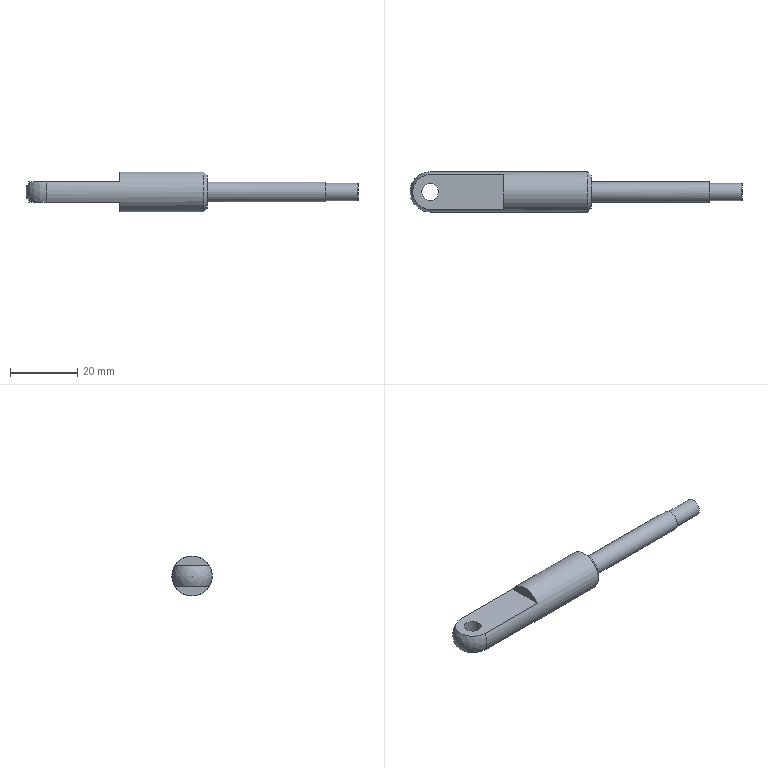Component | NX | SCREW_ROD | 1 solid | 14 faces | box 99 x 12 x 12 mm | volume 5834 mm3 | plane 7 | cylinder 4 | cone 2 | sphere 1 | commonest cylinder face diameters 12 x1 5 x1 6 x1 5.188 x1
STEP:
#1=CARTESIAN_POINT('',(0.,0.,0.));
#2=DIRECTION('',(0.,0.,1.));
#3=DIRECTION('',(1.,0.,0.));
#4=AXIS2_PLACEMENT_3D('',#1,#2,#3);
#5=CARTESIAN_POINT('',(22.3,-37.25,-16.5));
#6=VERTEX_POINT('',#5);
#7=CARTESIAN_POINT('',(22.3,-43.25,-16.5));
#8=DIRECTION('',(-1.,0.,0.));
#9=DIRECTION('',(0.,1.,0.));
#10=AXIS2_PLACEMENT_3D('',#7,#8,#9);
#11=CIRCLE('',#10,6.);
#12=CARTESIAN_POINT('',(-30.7,-43.25,-16.5));
#13=DIRECTION('',(1.,0.,0.));
#14=DIRECTION('',(0.,1.,0.));
#15=AXIS2_PLACEMENT_3D('',#12,#13,#14);
#16=CYLINDRICAL_SURFACE('',#15,6.);
#17=CARTESIAN_POINT('',(6.283,53.));
#18=DIRECTION('',(-1.,0.));
#19=VECTOR('',#18,1.);
#20=LINE('',#17,#19);
#21=(GEOMETRIC_REPRESENTATION_CONTEXT(2)PARAMETRIC_REPRESENTATION_CONTEXT()REPRESENTATION_CONTEXT('',''));
#22=DEFINITIONAL_REPRESENTATION('',(#20),#21);
#23=PCURVE('',#16,#22);
#24=CARTESIAN_POINT('',(23.3,-43.25,-16.5));
#25=DIRECTION('',(-1.,0.,0.));
#26=DIRECTION('',(0.,-1.,0.));
#27=AXIS2_PLACEMENT_3D('',#24,#25,#26);
#28=CONICAL_SURFACE('',#27,5.,0.7854);
#29=CARTESIAN_POINT('',(3.142,1.));
#30=DIRECTION('',(1.,0.));
#31=VECTOR('',#30,1.);
#32=LINE('',#29,#31);
#33=(GEOMETRIC_REPRESENTATION_CONTEXT(2)PARAMETRIC_REPRESENTATION_CONTEXT()REPRESENTATION_CONTEXT('',''));
#34=DEFINITIONAL_REPRESENTATION('',(#32),#33);
#35=PCURVE('',#28,#34);
#36=SURFACE_CURVE('',#11,(#23,#35),.PCURVE_S1.);
#37=EDGE_CURVE('',#6,#6,#36,.T.);
#38=ORIENTED_EDGE('',*,*,#37,.T.);
#39=CARTESIAN_POINT('',(-24.7,-37.25,-16.5));
#40=VERTEX_POINT('',#39);
#41=CARTESIAN_POINT('',(-24.7,-37.25,-16.5));
#42=CARTESIAN_POINT('',(22.3,-37.25,-16.5));
#43=B_SPLINE_CURVE_WITH_KNOTS('',1,(#41,#42),.UNSPECIFIED.,.F.,.F.,(2,2),(6.,53.),.PIECEWISE_BEZIER_KNOTS.);
#44=CARTESIAN_POINT('',(0.,0.));
#45=DIRECTION('',(0.,1.));
#46=VECTOR('',#45,1.);
#47=LINE('',#44,#46);
#48=(GEOMETRIC_REPRESENTATION_CONTEXT(2)PARAMETRIC_REPRESENTATION_CONTEXT()REPRESENTATION_CONTEXT('',''));
#49=DEFINITIONAL_REPRESENTATION('',(#47),#48);
#50=PCURVE('',#16,#49);
#51=CARTESIAN_POINT('',(6.283,0.));
#52=DIRECTION('',(0.,1.));
#53=VECTOR('',#52,1.);
#54=LINE('',#51,#53);
#55=(GEOMETRIC_REPRESENTATION_CONTEXT(2)PARAMETRIC_REPRESENTATION_CONTEXT()REPRESENTATION_CONTEXT('',''));
#56=DEFINITIONAL_REPRESENTATION('',(#54),#55);
#57=PCURVE('',#16,#56);
#58=SEAM_CURVE('',#43,(#50,#57),.PCURVE_S1.);
#59=EDGE_CURVE('',#40,#6,#58,.T.);
#60=ORIENTED_EDGE('',*,*,#59,.F.);
#61=CARTESIAN_POINT('',(-24.7,-38.054,-13.5));
#62=VERTEX_POINT('',#61);
#63=CARTESIAN_POINT('',(-24.7,-43.25,-16.5));
#64=DIRECTION('',(1.,0.,0.));
#65=DIRECTION('',(0.,1.,0.));
#66=AXIS2_PLACEMENT_3D('',#63,#64,#65);
#67=CIRCLE('',#66,6.);
#68=CARTESIAN_POINT('',(-6.283,6.));
#69=DIRECTION('',(1.,0.));
#70=VECTOR('',#69,1.);
#71=LINE('',#68,#70);
#72=(GEOMETRIC_REPRESENTATION_CONTEXT(2)PARAMETRIC_REPRESENTATION_CONTEXT()REPRESENTATION_CONTEXT('',''));
#73=DEFINITIONAL_REPRESENTATION('',(#71),#72);
#74=PCURVE('',#16,#73);
#75=CARTESIAN_POINT('',(-24.7,-43.25,-16.5));
#76=DIRECTION('',(1.,0.,0.));
#77=DIRECTION('',(0.,1.,0.));
#78=AXIS2_PLACEMENT_3D('',#75,#76,#77);
#79=SPHERICAL_SURFACE('',#78,6.);
#80=CARTESIAN_POINT('',(-6.283,0.));
#81=DIRECTION('',(1.,0.));
#82=VECTOR('',#81,1.);
#83=LINE('',#80,#82);
#84=(GEOMETRIC_REPRESENTATION_CONTEXT(2)PARAMETRIC_REPRESENTATION_CONTEXT()REPRESENTATION_CONTEXT('',''));
#85=DEFINITIONAL_REPRESENTATION('',(#83),#84);
#86=PCURVE('',#79,#85);
#87=SURFACE_CURVE('',#67,(#74,#86),.PCURVE_S1.);
#88=EDGE_CURVE('',#40,#62,#87,.T.);
#89=ORIENTED_EDGE('',*,*,#88,.T.);
#90=CARTESIAN_POINT('',(-2.7,-38.054,-13.5));
#91=VERTEX_POINT('',#90);
#92=CARTESIAN_POINT('',(-30.7,-38.054,-13.5));
#93=DIRECTION('',(-1.,0.,0.));
#94=VECTOR('',#93,1.);
#95=LINE('',#92,#94);
#96=CARTESIAN_POINT('',(0.5236,0.));
#97=DIRECTION('',(0.,-1.));
#98=VECTOR('',#97,1.);
#99=LINE('',#96,#98);
#100=(GEOMETRIC_REPRESENTATION_CONTEXT(2)PARAMETRIC_REPRESENTATION_CONTEXT()REPRESENTATION_CONTEXT('',''));
#101=DEFINITIONAL_REPRESENTATION('',(#99),#100);
#102=PCURVE('',#16,#101);
#103=CARTESIAN_POINT('',(-36.7,-55.75,-13.5));
#104=DIRECTION('',(0.,-0.,-1.));
#105=DIRECTION('',(0.,1.,-0.));
#106=AXIS2_PLACEMENT_3D('',#103,#104,#105);
#107=PLANE('',#106);
#108=CARTESIAN_POINT('',(17.696,6.));
#109=DIRECTION('',(0.,-1.));
#110=VECTOR('',#109,1.);
#111=LINE('',#108,#110);
#112=(GEOMETRIC_REPRESENTATION_CONTEXT(2)PARAMETRIC_REPRESENTATION_CONTEXT()REPRESENTATION_CONTEXT('',''));
#113=DEFINITIONAL_REPRESENTATION('',(#111),#112);
#114=PCURVE('',#107,#113);
#115=SURFACE_CURVE('',#95,(#102,#114),.PCURVE_S1.);
#116=EDGE_CURVE('',#91,#62,#115,.T.);
#117=ORIENTED_EDGE('',*,*,#116,.F.);
#118=CARTESIAN_POINT('',(-2.7,-48.446,-13.5));
#119=VERTEX_POINT('',#118);
#120=CARTESIAN_POINT('',(-2.7,-43.25,-16.5));
#121=DIRECTION('',(-1.,0.,0.));
#122=DIRECTION('',(0.,1.,0.));
#123=AXIS2_PLACEMENT_3D('',#120,#121,#122);
#124=CIRCLE('',#123,6.);
#125=CARTESIAN_POINT('',(6.283,28.));
#126=DIRECTION('',(-1.,0.));
#127=VECTOR('',#126,1.);
#128=LINE('',#125,#127);
#129=(GEOMETRIC_REPRESENTATION_CONTEXT(2)PARAMETRIC_REPRESENTATION_CONTEXT()REPRESENTATION_CONTEXT('',''));
#130=DEFINITIONAL_REPRESENTATION('',(#128),#129);
#131=PCURVE('',#16,#130);
#132=CARTESIAN_POINT('',(-2.7,-43.25,-16.5));
#133=DIRECTION('',(1.,0.,0.));
#134=DIRECTION('',(0.,1.,0.));
#135=AXIS2_PLACEMENT_3D('',#132,#133,#134);
#136=PLANE('',#135);
#137=CARTESIAN_POINT('',(6.,0.));
#138=CARTESIAN_POINT('',(6.,-10.392));
#139=CARTESIAN_POINT('',(-3.,-5.196));
#140=CARTESIAN_POINT('',(-12.,-0.));
#141=CARTESIAN_POINT('',(-3.,5.196));
#142=CARTESIAN_POINT('',(6.,10.392));
#143=CARTESIAN_POINT('',(6.,0.));
#144=(BOUNDED_CURVE()B_SPLINE_CURVE(2,(#137,#138,#139,#140,#141,#142,#143),.UNSPECIFIED.,.T.,.F.)B_SPLINE_CURVE_WITH_KNOTS((1,2,2,2,2,1),(-2.094,0.,2.094,4.189,6.283,8.378),.UNSPECIFIED.)CURVE()GEOMETRIC_REPRESENTATION_ITEM()RATIONAL_B_SPLINE_CURVE((1.,0.5,1.,0.5,1.,0.5,1.))REPRESENTATION_ITEM(''));
#145=(GEOMETRIC_REPRESENTATION_CONTEXT(2)PARAMETRIC_REPRESENTATION_CONTEXT()REPRESENTATION_CONTEXT('',''));
#146=DEFINITIONAL_REPRESENTATION('',(#144),#145);
#147=PCURVE('',#136,#146);
#148=SURFACE_CURVE('',#124,(#131,#147),.PCURVE_S1.);
#149=EDGE_CURVE('',#119,#91,#148,.T.);
#150=ORIENTED_EDGE('',*,*,#149,.F.);
#151=CARTESIAN_POINT('',(-24.7,-48.446,-13.5));
#152=VERTEX_POINT('',#151);
#153=CARTESIAN_POINT('',(-30.7,-48.446,-13.5));
#154=DIRECTION('',(1.,0.,0.));
#155=VECTOR('',#154,1.);
#156=LINE('',#153,#155);
#157=CARTESIAN_POINT('',(2.618,0.));
#158=DIRECTION('',(0.,1.));
#159=VECTOR('',#158,1.);
#160=LINE('',#157,#159);
#161=(GEOMETRIC_REPRESENTATION_CONTEXT(2)PARAMETRIC_REPRESENTATION_CONTEXT()REPRESENTATION_CONTEXT('',''));
#162=DEFINITIONAL_REPRESENTATION('',(#160),#161);
#163=PCURVE('',#16,#162);
#164=CARTESIAN_POINT('',(7.304,6.));
#165=DIRECTION('',(0.,1.));
#166=VECTOR('',#165,1.);
#167=LINE('',#164,#166);
#168=(GEOMETRIC_REPRESENTATION_CONTEXT(2)PARAMETRIC_REPRESENTATION_CONTEXT()REPRESENTATION_CONTEXT('',''));
#169=DEFINITIONAL_REPRESENTATION('',(#167),#168);
#170=PCURVE('',#107,#169);
#171=SURFACE_CURVE('',#156,(#163,#170),.PCURVE_S1.);
#172=EDGE_CURVE('',#152,#119,#171,.T.);
#173=ORIENTED_EDGE('',*,*,#172,.F.);
#174=CARTESIAN_POINT('',(-24.7,-48.446,-19.5));
#175=VERTEX_POINT('',#174);
#176=CARTESIAN_POINT('',(-24.7,-43.25,-16.5));
#177=DIRECTION('',(1.,0.,0.));
#178=DIRECTION('',(0.,1.,0.));
#179=AXIS2_PLACEMENT_3D('',#176,#177,#178);
#180=CIRCLE('',#179,6.);
#181=CARTESIAN_POINT('',(0.,6.));
#182=DIRECTION('',(1.,0.));
#183=VECTOR('',#182,1.);
#184=LINE('',#181,#183);
#185=(GEOMETRIC_REPRESENTATION_CONTEXT(2)PARAMETRIC_REPRESENTATION_CONTEXT()REPRESENTATION_CONTEXT('',''));
#186=DEFINITIONAL_REPRESENTATION('',(#184),#185);
#187=PCURVE('',#16,#186);
#188=CARTESIAN_POINT('',(0.,0.));
#189=DIRECTION('',(1.,0.));
#190=VECTOR('',#189,1.);
#191=LINE('',#188,#190);
#192=(GEOMETRIC_REPRESENTATION_CONTEXT(2)PARAMETRIC_REPRESENTATION_CONTEXT()REPRESENTATION_CONTEXT('',''));
#193=DEFINITIONAL_REPRESENTATION('',(#191),#192);
#194=PCURVE('',#79,#193);
#195=SURFACE_CURVE('',#180,(#187,#194),.PCURVE_S1.);
#196=EDGE_CURVE('',#152,#175,#195,.T.);
#197=ORIENTED_EDGE('',*,*,#196,.T.);
#198=CARTESIAN_POINT('',(-2.7,-48.446,-19.5));
#199=VERTEX_POINT('',#198);
#200=CARTESIAN_POINT('',(-30.7,-48.446,-19.5));
#201=DIRECTION('',(-1.,0.,0.));
#202=VECTOR('',#201,1.);
#203=LINE('',#200,#202);
#204=CARTESIAN_POINT('',(3.665,0.));
#205=DIRECTION('',(0.,-1.));
#206=VECTOR('',#205,1.);
#207=LINE('',#204,#206);
#208=(GEOMETRIC_REPRESENTATION_CONTEXT(2)PARAMETRIC_REPRESENTATION_CONTEXT()REPRESENTATION_CONTEXT('',''));
#209=DEFINITIONAL_REPRESENTATION('',(#207),#208);
#210=PCURVE('',#16,#209);
#211=CARTESIAN_POINT('',(-36.7,-32.25,-19.5));
#212=DIRECTION('',(0.,-0.,1.));
#213=DIRECTION('',(0.,-1.,-0.));
#214=AXIS2_PLACEMENT_3D('',#211,#212,#213);
#215=PLANE('',#214);
#216=CARTESIAN_POINT('',(16.196,6.));
#217=DIRECTION('',(0.,-1.));
#218=VECTOR('',#217,1.);
#219=LINE('',#216,#218);
#220=(GEOMETRIC_REPRESENTATION_CONTEXT(2)PARAMETRIC_REPRESENTATION_CONTEXT()REPRESENTATION_CONTEXT('',''));
#221=DEFINITIONAL_REPRESENTATION('',(#219),#220);
#222=PCURVE('',#215,#221);
#223=SURFACE_CURVE('',#203,(#210,#222),.PCURVE_S1.);
#224=EDGE_CURVE('',#199,#175,#223,.T.);
#225=ORIENTED_EDGE('',*,*,#224,.F.);
#226=CARTESIAN_POINT('',(-2.7,-38.054,-19.5));
#227=VERTEX_POINT('',#226);
#228=CARTESIAN_POINT('',(-2.7,-43.25,-16.5));
#229=DIRECTION('',(-1.,0.,0.));
#230=DIRECTION('',(0.,1.,0.));
#231=AXIS2_PLACEMENT_3D('',#228,#229,#230);
#232=CIRCLE('',#231,6.);
#233=CARTESIAN_POINT('',(6.283,28.));
#234=DIRECTION('',(-1.,0.));
#235=VECTOR('',#234,1.);
#236=LINE('',#233,#235);
#237=(GEOMETRIC_REPRESENTATION_CONTEXT(2)PARAMETRIC_REPRESENTATION_CONTEXT()REPRESENTATION_CONTEXT('',''));
#238=DEFINITIONAL_REPRESENTATION('',(#236),#237);
#239=PCURVE('',#16,#238);
#240=CARTESIAN_POINT('',(-2.7,-43.25,-16.5));
#241=DIRECTION('',(1.,0.,0.));
#242=DIRECTION('',(0.,1.,0.));
#243=AXIS2_PLACEMENT_3D('',#240,#241,#242);
#244=PLANE('',#243);
#245=CARTESIAN_POINT('',(6.,0.));
#246=CARTESIAN_POINT('',(6.,-10.392));
#247=CARTESIAN_POINT('',(-3.,-5.196));
#248=CARTESIAN_POINT('',(-12.,-0.));
#249=CARTESIAN_POINT('',(-3.,5.196));
#250=CARTESIAN_POINT('',(6.,10.392));
#251=CARTESIAN_POINT('',(6.,0.));
#252=(BOUNDED_CURVE()B_SPLINE_CURVE(2,(#245,#246,#247,#248,#249,#250,#251),.UNSPECIFIED.,.T.,.F.)B_SPLINE_CURVE_WITH_KNOTS((1,2,2,2,2,1),(-2.094,0.,2.094,4.189,6.283,8.378),.UNSPECIFIED.)CURVE()GEOMETRIC_REPRESENTATION_ITEM()RATIONAL_B_SPLINE_CURVE((1.,0.5,1.,0.5,1.,0.5,1.))REPRESENTATION_ITEM(''));
#253=(GEOMETRIC_REPRESENTATION_CONTEXT(2)PARAMETRIC_REPRESENTATION_CONTEXT()REPRESENTATION_CONTEXT('',''));
#254=DEFINITIONAL_REPRESENTATION('',(#252),#253);
#255=PCURVE('',#244,#254);
#256=SURFACE_CURVE('',#232,(#239,#255),.PCURVE_S1.);
#257=EDGE_CURVE('',#227,#199,#256,.T.);
#258=ORIENTED_EDGE('',*,*,#257,.F.);
#259=CARTESIAN_POINT('',(-24.7,-38.054,-19.5));
#260=VERTEX_POINT('',#259);
#261=CARTESIAN_POINT('',(-30.7,-38.054,-19.5));
#262=DIRECTION('',(1.,0.,0.));
#263=VECTOR('',#262,1.);
#264=LINE('',#261,#263);
#265=CARTESIAN_POINT('',(5.76,0.));
#266=DIRECTION('',(0.,1.));
#267=VECTOR('',#266,1.);
#268=LINE('',#265,#267);
#269=(GEOMETRIC_REPRESENTATION_CONTEXT(2)PARAMETRIC_REPRESENTATION_CONTEXT()REPRESENTATION_CONTEXT('',''));
#270=DEFINITIONAL_REPRESENTATION('',(#268),#269);
#271=PCURVE('',#16,#270);
#272=CARTESIAN_POINT('',(5.804,6.));
#273=DIRECTION('',(0.,1.));
#274=VECTOR('',#273,1.);
#275=LINE('',#272,#274);
#276=(GEOMETRIC_REPRESENTATION_CONTEXT(2)PARAMETRIC_REPRESENTATION_CONTEXT()REPRESENTATION_CONTEXT('',''));
#277=DEFINITIONAL_REPRESENTATION('',(#275),#276);
#278=PCURVE('',#215,#277);
#279=SURFACE_CURVE('',#264,(#271,#278),.PCURVE_S1.);
#280=EDGE_CURVE('',#260,#227,#279,.T.);
#281=ORIENTED_EDGE('',*,*,#280,.F.);
#282=CARTESIAN_POINT('',(-24.7,-43.25,-16.5));
#283=DIRECTION('',(1.,0.,0.));
#284=DIRECTION('',(0.,1.,0.));
#285=AXIS2_PLACEMENT_3D('',#282,#283,#284);
#286=CIRCLE('',#285,6.);
#287=CARTESIAN_POINT('',(0.,6.));
#288=DIRECTION('',(1.,0.));
#289=VECTOR('',#288,1.);
#290=LINE('',#287,#289);
#291=(GEOMETRIC_REPRESENTATION_CONTEXT(2)PARAMETRIC_REPRESENTATION_CONTEXT()REPRESENTATION_CONTEXT('',''));
#292=DEFINITIONAL_REPRESENTATION('',(#290),#291);
#293=PCURVE('',#16,#292);
#294=CARTESIAN_POINT('',(5.76,0.));
#295=CARTESIAN_POINT('',(5.768,0.));
#296=CARTESIAN_POINT('',(5.783,0.));
#297=CARTESIAN_POINT('',(5.807,0.));
#298=CARTESIAN_POINT('',(5.831,0.));
#299=CARTESIAN_POINT('',(5.855,0.));
#300=CARTESIAN_POINT('',(5.879,0.));
#301=CARTESIAN_POINT('',(5.902,0.));
#302=CARTESIAN_POINT('',(5.926,0.));
#303=CARTESIAN_POINT('',(5.95,0.));
#304=CARTESIAN_POINT('',(5.974,0.));
#305=CARTESIAN_POINT('',(5.998,0.));
#306=CARTESIAN_POINT('',(6.021,0.));
#307=CARTESIAN_POINT('',(6.045,0.));
#308=CARTESIAN_POINT('',(6.069,0.));
#309=CARTESIAN_POINT('',(6.093,0.));
#310=CARTESIAN_POINT('',(6.117,0.));
#311=CARTESIAN_POINT('',(6.14,0.));
#312=CARTESIAN_POINT('',(6.164,0.));
#313=CARTESIAN_POINT('',(6.188,0.));
#314=CARTESIAN_POINT('',(6.212,0.));
#315=CARTESIAN_POINT('',(6.236,0.));
#316=CARTESIAN_POINT('',(6.259,0.));
#317=CARTESIAN_POINT('',(6.275,0.));
#318=CARTESIAN_POINT('',(6.283,0.));
#319=B_SPLINE_CURVE_WITH_KNOTS('',3,(#294,#295,#296,#297,#298,#299,#300,#301,#302,#303,#304,#305,#306,#307,#308,#309,#310,#311,#312,#313,#314,#315,#316,#317,#318),.UNSPECIFIED.,.F.,.F.,(4,1,1,1,1,1,1,1,1,1,1,1,1,1,1,1,1,1,1,1,1,1,4),(5.76,5.783,5.807,5.831,5.855,5.879,5.902,5.926,5.95,5.974,5.998,6.021,6.045,6.069,6.093,6.117,6.14,6.164,6.188,6.212,6.236,6.259,6.283),.QUASI_UNIFORM_KNOTS.);
#320=(GEOMETRIC_REPRESENTATION_CONTEXT(2)PARAMETRIC_REPRESENTATION_CONTEXT()REPRESENTATION_CONTEXT('',''));
#321=DEFINITIONAL_REPRESENTATION('',(#319),#320);
#322=PCURVE('',#79,#321);
#323=SURFACE_CURVE('',#286,(#293,#322),.PCURVE_S1.);
#324=EDGE_CURVE('',#260,#40,#323,.T.);
#325=ORIENTED_EDGE('',*,*,#324,.T.);
#326=ORIENTED_EDGE('',*,*,#59,.T.);
#327=EDGE_LOOP('',(#38,#60,#89,#117,#150,#173,#197,#225,#258,#281,#325,#326));
#328=FACE_BOUND('',#327,.T.);
#329=ADVANCED_FACE('',(#328),#16,.T.);
#330=CARTESIAN_POINT('',(23.3,-38.25,-16.5));
#331=VERTEX_POINT('',#330);
#332=CARTESIAN_POINT('',(23.3,-43.25,-16.5));
#333=DIRECTION('',(1.,0.,0.));
#334=DIRECTION('',(0.,1.,0.));
#335=AXIS2_PLACEMENT_3D('',#332,#333,#334);
#336=CIRCLE('',#335,5.);
#337=CARTESIAN_POINT('',(23.3,-43.25,-16.5));
#338=DIRECTION('',(1.,0.,0.));
#339=DIRECTION('',(0.,1.,0.));
#340=AXIS2_PLACEMENT_3D('',#337,#338,#339);
#341=PLANE('',#340);
#342=CARTESIAN_POINT('',(0.,0.));
#343=DIRECTION('',(1.,0.));
#344=AXIS2_PLACEMENT_2D('',#342,#343);
#345=CIRCLE('',#344,5.);
#346=(GEOMETRIC_REPRESENTATION_CONTEXT(2)PARAMETRIC_REPRESENTATION_CONTEXT()REPRESENTATION_CONTEXT('',''));
#347=DEFINITIONAL_REPRESENTATION('',(#345),#346);
#348=PCURVE('',#341,#347);
#349=CARTESIAN_POINT('',(9.425,0.));
#350=DIRECTION('',(-1.,0.));
#351=VECTOR('',#350,1.);
#352=LINE('',#349,#351);
#353=(GEOMETRIC_REPRESENTATION_CONTEXT(2)PARAMETRIC_REPRESENTATION_CONTEXT()REPRESENTATION_CONTEXT('',''));
#354=DEFINITIONAL_REPRESENTATION('',(#352),#353);
#355=PCURVE('',#28,#354);
#356=SURFACE_CURVE('',#336,(#348,#355),.PCURVE_S1.);
#357=EDGE_CURVE('',#331,#331,#356,.T.);
#358=ORIENTED_EDGE('',*,*,#357,.T.);
#359=EDGE_LOOP('',(#358));
#360=FACE_BOUND('',#359,.T.);
#361=CARTESIAN_POINT('',(23.3,-43.25,-13.5));
#362=VERTEX_POINT('',#361);
#363=CARTESIAN_POINT('',(23.3,-46.25,-16.5));
#364=VERTEX_POINT('',#363);
#365=CARTESIAN_POINT('',(23.3,-43.25,-16.5));
#366=DIRECTION('',(1.,0.,0.));
#367=DIRECTION('',(0.,0.,1.));
#368=AXIS2_PLACEMENT_3D('',#365,#366,#367);
#369=CIRCLE('',#368,3.);
#370=CARTESIAN_POINT('',(0.,0.));
#371=DIRECTION('',(0.,1.));
#372=AXIS2_PLACEMENT_2D('',#370,#371);
#373=CIRCLE('',#372,3.);
#374=(GEOMETRIC_REPRESENTATION_CONTEXT(2)PARAMETRIC_REPRESENTATION_CONTEXT()REPRESENTATION_CONTEXT('',''));
#375=DEFINITIONAL_REPRESENTATION('',(#373),#374);
#376=PCURVE('',#341,#375);
#377=CARTESIAN_POINT('',(68.3,-43.25,-16.5));
#378=DIRECTION('',(-1.,0.,0.));
#379=DIRECTION('',(0.,-1.,0.));
#380=AXIS2_PLACEMENT_3D('',#377,#378,#379);
#381=CYLINDRICAL_SURFACE('',#380,3.);
#382=CARTESIAN_POINT('',(1.571,45.));
#383=DIRECTION('',(-1.,0.));
#384=VECTOR('',#383,1.);
#385=LINE('',#382,#384);
#386=(GEOMETRIC_REPRESENTATION_CONTEXT(2)PARAMETRIC_REPRESENTATION_CONTEXT()REPRESENTATION_CONTEXT('',''));
#387=DEFINITIONAL_REPRESENTATION('',(#385),#386);
#388=PCURVE('',#381,#387);
#389=SURFACE_CURVE('',#369,(#376,#388),.PCURVE_S1.);
#390=EDGE_CURVE('',#362,#364,#389,.T.);
#391=ORIENTED_EDGE('',*,*,#390,.F.);
#392=CARTESIAN_POINT('',(23.3,-43.25,-16.5));
#393=DIRECTION('',(1.,0.,0.));
#394=DIRECTION('',(0.,0.,1.));
#395=AXIS2_PLACEMENT_3D('',#392,#393,#394);
#396=CIRCLE('',#395,3.);
#397=CARTESIAN_POINT('',(0.,0.));
#398=DIRECTION('',(0.,1.));
#399=AXIS2_PLACEMENT_2D('',#397,#398);
#400=CIRCLE('',#399,3.);
#401=(GEOMETRIC_REPRESENTATION_CONTEXT(2)PARAMETRIC_REPRESENTATION_CONTEXT()REPRESENTATION_CONTEXT('',''));
#402=DEFINITIONAL_REPRESENTATION('',(#400),#401);
#403=PCURVE('',#341,#402);
#404=CARTESIAN_POINT('',(7.854,45.));
#405=DIRECTION('',(-1.,0.));
#406=VECTOR('',#405,1.);
#407=LINE('',#404,#406);
#408=(GEOMETRIC_REPRESENTATION_CONTEXT(2)PARAMETRIC_REPRESENTATION_CONTEXT()REPRESENTATION_CONTEXT('',''));
#409=DEFINITIONAL_REPRESENTATION('',(#407),#408);
#410=PCURVE('',#381,#409);
#411=SURFACE_CURVE('',#396,(#403,#410),.PCURVE_S1.);
#412=EDGE_CURVE('',#364,#362,#411,.T.);
#413=ORIENTED_EDGE('',*,*,#412,.F.);
#414=EDGE_LOOP('',(#391,#413));
#415=FACE_BOUND('',#414,.T.);
#416=ADVANCED_FACE('',(#360,#415),#341,.T.);
#417=CARTESIAN_POINT('',(-24.7,-43.25,-19.5));
#418=DIRECTION('',(0.,0.,-1.));
#419=DIRECTION('',(0.,-1.,-0.));
#420=AXIS2_PLACEMENT_3D('',#417,#418,#419);
#421=CIRCLE('',#420,5.196);
#422=CARTESIAN_POINT('',(3.665,0.));
#423=CARTESIAN_POINT('',(3.665,-0.04121));
#424=CARTESIAN_POINT('',(3.668,-0.1237));
#425=CARTESIAN_POINT('',(3.682,-0.2467));
#426=CARTESIAN_POINT('',(3.705,-0.3684));
#427=CARTESIAN_POINT('',(3.741,-0.4878));
#428=CARTESIAN_POINT('',(3.791,-0.6039));
#429=CARTESIAN_POINT('',(3.86,-0.7148));
#430=CARTESIAN_POINT('',(3.954,-0.8181));
#431=CARTESIAN_POINT('',(4.082,-0.91));
#432=CARTESIAN_POINT('',(4.251,-0.9849));
#433=CARTESIAN_POINT('',(4.465,-1.035));
#434=CARTESIAN_POINT('',(4.712,-1.053));
#435=CARTESIAN_POINT('',(4.96,-1.035));
#436=CARTESIAN_POINT('',(5.174,-0.9849));
#437=CARTESIAN_POINT('',(5.343,-0.91));
#438=CARTESIAN_POINT('',(5.47,-0.8181));
#439=CARTESIAN_POINT('',(5.565,-0.7148));
#440=CARTESIAN_POINT('',(5.634,-0.6039));
#441=CARTESIAN_POINT('',(5.684,-0.4878));
#442=CARTESIAN_POINT('',(5.72,-0.3684));
#443=CARTESIAN_POINT('',(5.743,-0.2467));
#444=CARTESIAN_POINT('',(5.757,-0.1237));
#445=CARTESIAN_POINT('',(5.76,-0.04121));
#446=CARTESIAN_POINT('',(5.76,0.));
#447=B_SPLINE_CURVE_WITH_KNOTS('',3,(#422,#423,#424,#425,#426,#427,#428,#429,#430,#431,#432,#433,#434,#435,#436,#437,#438,#439,#440,#441,#442,#443,#444,#445,#446),.UNSPECIFIED.,.F.,.F.,(4,1,1,1,1,1,1,1,1,1,1,1,1,1,1,1,1,1,1,1,1,1,4),(0.,0.1428,0.2856,0.4284,0.5712,0.714,0.8568,0.9996,1.142,1.285,1.428,1.571,1.714,1.856,1.999,2.142,2.285,2.428,2.57,2.713,2.856,2.999,3.142),.QUASI_UNIFORM_KNOTS.);
#448=(GEOMETRIC_REPRESENTATION_CONTEXT(2)PARAMETRIC_REPRESENTATION_CONTEXT()REPRESENTATION_CONTEXT('',''));
#449=DEFINITIONAL_REPRESENTATION('',(#447),#448);
#450=PCURVE('',#79,#449);
#451=CARTESIAN_POINT('',(16.196,12.));
#452=CARTESIAN_POINT('',(16.196,3.));
#453=CARTESIAN_POINT('',(8.402,7.5));
#454=CARTESIAN_POINT('',(0.6077,12.));
#455=CARTESIAN_POINT('',(8.402,16.5));
#456=CARTESIAN_POINT('',(16.196,21.));
#457=CARTESIAN_POINT('',(16.196,12.));
#458=(BOUNDED_CURVE()B_SPLINE_CURVE(2,(#451,#452,#453,#454,#455,#456,#457),.UNSPECIFIED.,.T.,.F.)B_SPLINE_CURVE_WITH_KNOTS((1,2,2,2,2,1),(-2.094,0.,2.094,4.189,6.283,8.378),.UNSPECIFIED.)CURVE()GEOMETRIC_REPRESENTATION_ITEM()RATIONAL_B_SPLINE_CURVE((1.,0.5,1.,0.5,1.,0.5,1.))REPRESENTATION_ITEM(''));
#459=(GEOMETRIC_REPRESENTATION_CONTEXT(2)PARAMETRIC_REPRESENTATION_CONTEXT()REPRESENTATION_CONTEXT('',''));
#460=DEFINITIONAL_REPRESENTATION('',(#458),#459);
#461=PCURVE('',#215,#460);
#462=SURFACE_CURVE('',#421,(#450,#461),.PCURVE_S1.);
#463=EDGE_CURVE('',#175,#260,#462,.T.);
#464=ORIENTED_EDGE('',*,*,#463,.F.);
#465=ORIENTED_EDGE('',*,*,#196,.F.);
#466=CARTESIAN_POINT('',(-24.7,-43.25,-13.5));
#467=DIRECTION('',(0.,0.,1.));
#468=DIRECTION('',(0.,1.,-0.));
#469=AXIS2_PLACEMENT_3D('',#466,#467,#468);
#470=CIRCLE('',#469,5.196);
#471=CARTESIAN_POINT('',(0.5236,0.));
#472=CARTESIAN_POINT('',(0.5237,-0.04121));
#473=CARTESIAN_POINT('',(0.5265,-0.1237));
#474=CARTESIAN_POINT('',(0.54,-0.2467));
#475=CARTESIAN_POINT('',(0.5636,-0.3684));
#476=CARTESIAN_POINT('',(0.599,-0.4878));
#477=CARTESIAN_POINT('',(0.6492,-0.6039));
#478=CARTESIAN_POINT('',(0.7184,-0.7148));
#479=CARTESIAN_POINT('',(0.8127,-0.8181));
#480=CARTESIAN_POINT('',(0.9401,-0.91));
#481=CARTESIAN_POINT('',(1.109,-0.9849));
#482=CARTESIAN_POINT('',(1.324,-1.035));
#483=CARTESIAN_POINT('',(1.571,-1.053));
#484=CARTESIAN_POINT('',(1.818,-1.035));
#485=CARTESIAN_POINT('',(2.032,-0.9849));
#486=CARTESIAN_POINT('',(2.201,-0.91));
#487=CARTESIAN_POINT('',(2.329,-0.8181));
#488=CARTESIAN_POINT('',(2.423,-0.7148));
#489=CARTESIAN_POINT('',(2.492,-0.6039));
#490=CARTESIAN_POINT('',(2.543,-0.4878));
#491=CARTESIAN_POINT('',(2.578,-0.3684));
#492=CARTESIAN_POINT('',(2.602,-0.2467));
#493=CARTESIAN_POINT('',(2.615,-0.1237));
#494=CARTESIAN_POINT('',(2.618,-0.04121));
#495=CARTESIAN_POINT('',(2.618,0.));
#496=B_SPLINE_CURVE_WITH_KNOTS('',3,(#471,#472,#473,#474,#475,#476,#477,#478,#479,#480,#481,#482,#483,#484,#485,#486,#487,#488,#489,#490,#491,#492,#493,#494,#495),.UNSPECIFIED.,.F.,.F.,(4,1,1,1,1,1,1,1,1,1,1,1,1,1,1,1,1,1,1,1,1,1,4),(0.,0.1428,0.2856,0.4284,0.5712,0.714,0.8568,0.9996,1.142,1.285,1.428,1.571,1.714,1.856,1.999,2.142,2.285,2.428,2.57,2.713,2.856,2.999,3.142),.QUASI_UNIFORM_KNOTS.);
#497=(GEOMETRIC_REPRESENTATION_CONTEXT(2)PARAMETRIC_REPRESENTATION_CONTEXT()REPRESENTATION_CONTEXT('',''));
#498=DEFINITIONAL_REPRESENTATION('',(#496),#497);
#499=PCURVE('',#79,#498);
#500=CARTESIAN_POINT('',(17.696,12.));
#501=CARTESIAN_POINT('',(17.696,3.));
#502=CARTESIAN_POINT('',(9.902,7.5));
#503=CARTESIAN_POINT('',(2.108,12.));
#504=CARTESIAN_POINT('',(9.902,16.5));
#505=CARTESIAN_POINT('',(17.696,21.));
#506=CARTESIAN_POINT('',(17.696,12.));
#507=(BOUNDED_CURVE()B_SPLINE_CURVE(2,(#500,#501,#502,#503,#504,#505,#506),.UNSPECIFIED.,.T.,.F.)B_SPLINE_CURVE_WITH_KNOTS((1,2,2,2,2,1),(-2.094,0.,2.094,4.189,6.283,8.378),.UNSPECIFIED.)CURVE()GEOMETRIC_REPRESENTATION_ITEM()RATIONAL_B_SPLINE_CURVE((1.,0.5,1.,0.5,1.,0.5,1.))REPRESENTATION_ITEM(''));
#508=(GEOMETRIC_REPRESENTATION_CONTEXT(2)PARAMETRIC_REPRESENTATION_CONTEXT()REPRESENTATION_CONTEXT('',''));
#509=DEFINITIONAL_REPRESENTATION('',(#507),#508);
#510=PCURVE('',#107,#509);
#511=SURFACE_CURVE('',#470,(#499,#510),.PCURVE_S1.);
#512=EDGE_CURVE('',#62,#152,#511,.T.);
#513=ORIENTED_EDGE('',*,*,#512,.F.);
#514=ORIENTED_EDGE('',*,*,#88,.F.);
#515=CARTESIAN_POINT('',(-30.7,-43.25,-16.5));
#516=VERTEX_POINT('',#515);
#517=CARTESIAN_POINT('',(-30.7,-43.25,-16.5));
#518=CARTESIAN_POINT('',(-30.7,-41.904,-16.5));
#519=CARTESIAN_POINT('',(-30.348,-40.557,-16.5));
#520=CARTESIAN_POINT('',(-29.643,-39.322,-16.5));
#521=CARTESIAN_POINT('',(-28.628,-38.307,-16.5));
#522=CARTESIAN_POINT('',(-27.393,-37.602,-16.5));
#523=CARTESIAN_POINT('',(-26.046,-37.25,-16.5));
#524=CARTESIAN_POINT('',(-24.7,-37.25,-16.5));
#525=B_SPLINE_CURVE_WITH_KNOTS('',7,(#517,#518,#519,#520,#521,#522,#523,#524),.UNSPECIFIED.,.F.,.F.,(8,8),(-1.571,0.),.PIECEWISE_BEZIER_KNOTS.);
#526=CARTESIAN_POINT('',(0.,0.));
#527=DIRECTION('',(0.,1.));
#528=VECTOR('',#527,1.);
#529=LINE('',#526,#528);
#530=(GEOMETRIC_REPRESENTATION_CONTEXT(2)PARAMETRIC_REPRESENTATION_CONTEXT()REPRESENTATION_CONTEXT('',''));
#531=DEFINITIONAL_REPRESENTATION('',(#529),#530);
#532=PCURVE('',#79,#531);
#533=CARTESIAN_POINT('',(6.283,0.));
#534=DIRECTION('',(0.,1.));
#535=VECTOR('',#534,1.);
#536=LINE('',#533,#535);
#537=(GEOMETRIC_REPRESENTATION_CONTEXT(2)PARAMETRIC_REPRESENTATION_CONTEXT()REPRESENTATION_CONTEXT('',''));
#538=DEFINITIONAL_REPRESENTATION('',(#536),#537);
#539=PCURVE('',#79,#538);
#540=SEAM_CURVE('',#525,(#532,#539),.PCURVE_S1.);
#541=EDGE_CURVE('',#516,#40,#540,.T.);
#542=ORIENTED_EDGE('',*,*,#541,.F.);
#543=ORIENTED_EDGE('',*,*,#541,.T.);
#544=ORIENTED_EDGE('',*,*,#324,.F.);
#545=EDGE_LOOP('',(#464,#465,#513,#514,#542,#543,#544));
#546=FACE_BOUND('',#545,.T.);
#547=ADVANCED_FACE('',(#546),#79,.T.);
#548=CARTESIAN_POINT('',(-24.7,-40.75,-13.5));
#549=VERTEX_POINT('',#548);
#550=CARTESIAN_POINT('',(-24.7,-45.75,-13.5));
#551=VERTEX_POINT('',#550);
#552=CARTESIAN_POINT('',(-24.7,-43.25,-13.5));
#553=DIRECTION('',(0.,-0.,-1.));
#554=DIRECTION('',(0.,1.,-0.));
#555=AXIS2_PLACEMENT_3D('',#552,#553,#554);
#556=CIRCLE('',#555,2.5);
#557=CARTESIAN_POINT('',(12.5,12.));
#558=DIRECTION('',(1.,0.));
#559=AXIS2_PLACEMENT_2D('',#557,#558);
#560=CIRCLE('',#559,2.5);
#561=(GEOMETRIC_REPRESENTATION_CONTEXT(2)PARAMETRIC_REPRESENTATION_CONTEXT()REPRESENTATION_CONTEXT('',''));
#562=DEFINITIONAL_REPRESENTATION('',(#560),#561);
#563=PCURVE('',#107,#562);
#564=CARTESIAN_POINT('',(-24.7,-43.25,-19.5));
#565=DIRECTION('',(0.,-0.,1.));
#566=DIRECTION('',(0.,-1.,-0.));
#567=AXIS2_PLACEMENT_3D('',#564,#565,#566);
#568=CYLINDRICAL_SURFACE('',#567,2.5);
#569=CARTESIAN_POINT('',(3.142,6.));
#570=DIRECTION('',(-1.,0.));
#571=VECTOR('',#570,1.);
#572=LINE('',#569,#571);
#573=(GEOMETRIC_REPRESENTATION_CONTEXT(2)PARAMETRIC_REPRESENTATION_CONTEXT()REPRESENTATION_CONTEXT('',''));
#574=DEFINITIONAL_REPRESENTATION('',(#572),#573);
#575=PCURVE('',#568,#574);
#576=SURFACE_CURVE('',#556,(#563,#575),.PCURVE_S1.);
#577=EDGE_CURVE('',#549,#551,#576,.T.);
#578=ORIENTED_EDGE('',*,*,#577,.T.);
#579=CARTESIAN_POINT('',(-24.7,-43.25,-13.5));
#580=DIRECTION('',(0.,-0.,-1.));
#581=DIRECTION('',(0.,1.,-0.));
#582=AXIS2_PLACEMENT_3D('',#579,#580,#581);
#583=CIRCLE('',#582,2.5);
#584=CARTESIAN_POINT('',(12.5,12.));
#585=DIRECTION('',(1.,0.));
#586=AXIS2_PLACEMENT_2D('',#584,#585);
#587=CIRCLE('',#586,2.5);
#588=(GEOMETRIC_REPRESENTATION_CONTEXT(2)PARAMETRIC_REPRESENTATION_CONTEXT()REPRESENTATION_CONTEXT('',''));
#589=DEFINITIONAL_REPRESENTATION('',(#587),#588);
#590=PCURVE('',#107,#589);
#591=CARTESIAN_POINT('',(9.425,6.));
#592=DIRECTION('',(-1.,0.));
#593=VECTOR('',#592,1.);
#594=LINE('',#591,#593);
#595=(GEOMETRIC_REPRESENTATION_CONTEXT(2)PARAMETRIC_REPRESENTATION_CONTEXT()REPRESENTATION_CONTEXT('',''));
#596=DEFINITIONAL_REPRESENTATION('',(#594),#595);
#597=PCURVE('',#568,#596);
#598=SURFACE_CURVE('',#583,(#590,#597),.PCURVE_S1.);
#599=EDGE_CURVE('',#551,#549,#598,.T.);
#600=ORIENTED_EDGE('',*,*,#599,.T.);
#601=EDGE_LOOP('',(#578,#600));
#602=FACE_BOUND('',#601,.T.);
#603=ORIENTED_EDGE('',*,*,#116,.T.);
#604=ORIENTED_EDGE('',*,*,#512,.T.);
#605=ORIENTED_EDGE('',*,*,#172,.T.);
#606=CARTESIAN_POINT('',(-2.7,-55.75,-13.5));
#607=DIRECTION('',(0.,-1.,0.));
#608=VECTOR('',#607,1.);
#609=LINE('',#606,#608);
#610=CARTESIAN_POINT('',(0.,34.));
#611=DIRECTION('',(-1.,0.));
#612=VECTOR('',#611,1.);
#613=LINE('',#610,#612);
#614=(GEOMETRIC_REPRESENTATION_CONTEXT(2)PARAMETRIC_REPRESENTATION_CONTEXT()REPRESENTATION_CONTEXT('',''));
#615=DEFINITIONAL_REPRESENTATION('',(#613),#614);
#616=PCURVE('',#107,#615);
#617=CARTESIAN_POINT('',(-12.5,3.));
#618=DIRECTION('',(-1.,0.));
#619=VECTOR('',#618,1.);
#620=LINE('',#617,#619);
#621=(GEOMETRIC_REPRESENTATION_CONTEXT(2)PARAMETRIC_REPRESENTATION_CONTEXT()REPRESENTATION_CONTEXT('',''));
#622=DEFINITIONAL_REPRESENTATION('',(#620),#621);
#623=PCURVE('',#136,#622);
#624=SURFACE_CURVE('',#609,(#616,#623),.PCURVE_S1.);
#625=EDGE_CURVE('',#91,#119,#624,.T.);
#626=ORIENTED_EDGE('',*,*,#625,.F.);
#627=EDGE_LOOP('',(#603,#604,#605,#626));
#628=FACE_BOUND('',#627,.T.);
#629=ADVANCED_FACE('',(#602,#628),#107,.F.);
#630=ORIENTED_EDGE('',*,*,#149,.T.);
#631=ORIENTED_EDGE('',*,*,#625,.T.);
#632=EDGE_LOOP('',(#630,#631));
#633=FACE_BOUND('',#632,.T.);
#634=ADVANCED_FACE('',(#633),#136,.F.);
#635=CARTESIAN_POINT('',(-24.7,-45.75,-19.5));
#636=VERTEX_POINT('',#635);
#637=CARTESIAN_POINT('',(-24.7,-43.25,-19.5));
#638=DIRECTION('',(0.,-0.,1.));
#639=DIRECTION('',(0.,-1.,-0.));
#640=AXIS2_PLACEMENT_3D('',#637,#638,#639);
#641=CIRCLE('',#640,2.5);
#642=CARTESIAN_POINT('',(11.,12.));
#643=DIRECTION('',(1.,0.));
#644=AXIS2_PLACEMENT_2D('',#642,#643);
#645=CIRCLE('',#644,2.5);
#646=(GEOMETRIC_REPRESENTATION_CONTEXT(2)PARAMETRIC_REPRESENTATION_CONTEXT()REPRESENTATION_CONTEXT('',''));
#647=DEFINITIONAL_REPRESENTATION('',(#645),#646);
#648=PCURVE('',#215,#647);
#649=CARTESIAN_POINT('',(0.,0.));
#650=DIRECTION('',(1.,0.));
#651=VECTOR('',#650,1.);
#652=LINE('',#649,#651);
#653=(GEOMETRIC_REPRESENTATION_CONTEXT(2)PARAMETRIC_REPRESENTATION_CONTEXT()REPRESENTATION_CONTEXT('',''));
#654=DEFINITIONAL_REPRESENTATION('',(#652),#653);
#655=PCURVE('',#568,#654);
#656=SURFACE_CURVE('',#641,(#648,#655),.PCURVE_S1.);
#657=EDGE_CURVE('',#636,#636,#656,.T.);
#658=ORIENTED_EDGE('',*,*,#657,.T.);
#659=EDGE_LOOP('',(#658));
#660=FACE_BOUND('',#659,.T.);
#661=ORIENTED_EDGE('',*,*,#224,.T.);
#662=ORIENTED_EDGE('',*,*,#463,.T.);
#663=ORIENTED_EDGE('',*,*,#280,.T.);
#664=CARTESIAN_POINT('',(-2.7,-32.25,-19.5));
#665=DIRECTION('',(0.,1.,0.));
#666=VECTOR('',#665,1.);
#667=LINE('',#664,#666);
#668=CARTESIAN_POINT('',(0.,34.));
#669=DIRECTION('',(-1.,0.));
#670=VECTOR('',#669,1.);
#671=LINE('',#668,#670);
#672=(GEOMETRIC_REPRESENTATION_CONTEXT(2)PARAMETRIC_REPRESENTATION_CONTEXT()REPRESENTATION_CONTEXT('',''));
#673=DEFINITIONAL_REPRESENTATION('',(#671),#672);
#674=PCURVE('',#215,#673);
#675=CARTESIAN_POINT('',(11.,-3.));
#676=DIRECTION('',(1.,0.));
#677=VECTOR('',#676,1.);
#678=LINE('',#675,#677);
#679=(GEOMETRIC_REPRESENTATION_CONTEXT(2)PARAMETRIC_REPRESENTATION_CONTEXT()REPRESENTATION_CONTEXT('',''));
#680=DEFINITIONAL_REPRESENTATION('',(#678),#679);
#681=PCURVE('',#244,#680);
#682=SURFACE_CURVE('',#667,(#674,#681),.PCURVE_S1.);
#683=EDGE_CURVE('',#199,#227,#682,.T.);
#684=ORIENTED_EDGE('',*,*,#683,.F.);
#685=EDGE_LOOP('',(#661,#662,#663,#684));
#686=FACE_BOUND('',#685,.T.);
#687=ADVANCED_FACE('',(#660,#686),#215,.F.);
#688=ORIENTED_EDGE('',*,*,#257,.T.);
#689=ORIENTED_EDGE('',*,*,#683,.T.);
#690=EDGE_LOOP('',(#688,#689));
#691=FACE_BOUND('',#690,.T.);
#692=ADVANCED_FACE('',(#691),#244,.F.);
#693=ORIENTED_EDGE('',*,*,#657,.T.);
#694=CARTESIAN_POINT('',(-24.7,-45.75,-19.5));
#695=CARTESIAN_POINT('',(-24.7,-45.75,-13.5));
#696=B_SPLINE_CURVE_WITH_KNOTS('',1,(#694,#695),.UNSPECIFIED.,.F.,.F.,(2,2),(0.,6.),.PIECEWISE_BEZIER_KNOTS.);
#697=CARTESIAN_POINT('',(6.283,0.));
#698=DIRECTION('',(0.,1.));
#699=VECTOR('',#698,1.);
#700=LINE('',#697,#699);
#701=(GEOMETRIC_REPRESENTATION_CONTEXT(2)PARAMETRIC_REPRESENTATION_CONTEXT()REPRESENTATION_CONTEXT('',''));
#702=DEFINITIONAL_REPRESENTATION('',(#700),#701);
#703=PCURVE('',#568,#702);
#704=CARTESIAN_POINT('',(0.,0.));
#705=DIRECTION('',(0.,1.));
#706=VECTOR('',#705,1.);
#707=LINE('',#704,#706);
#708=(GEOMETRIC_REPRESENTATION_CONTEXT(2)PARAMETRIC_REPRESENTATION_CONTEXT()REPRESENTATION_CONTEXT('',''));
#709=DEFINITIONAL_REPRESENTATION('',(#707),#708);
#710=PCURVE('',#568,#709);
#711=SEAM_CURVE('',#696,(#703,#710),.PCURVE_S1.);
#712=EDGE_CURVE('',#636,#551,#711,.T.);
#713=ORIENTED_EDGE('',*,*,#712,.T.);
#714=ORIENTED_EDGE('',*,*,#599,.T.);
#715=ORIENTED_EDGE('',*,*,#577,.T.);
#716=ORIENTED_EDGE('',*,*,#712,.F.);
#717=EDGE_LOOP('',(#693,#713,#714,#715,#716));
#718=FACE_BOUND('',#717,.F.);
#719=ADVANCED_FACE('',(#718),#568,.F.);
#720=CARTESIAN_POINT('',(58.6,-46.25,-16.5));
#721=VERTEX_POINT('',#720);
#722=CARTESIAN_POINT('',(58.6,-43.25,-16.5));
#723=DIRECTION('',(-1.,0.,0.));
#724=DIRECTION('',(0.,-1.,0.));
#725=AXIS2_PLACEMENT_3D('',#722,#723,#724);
#726=CIRCLE('',#725,3.);
#727=CARTESIAN_POINT('',(0.,9.7));
#728=DIRECTION('',(1.,0.));
#729=VECTOR('',#728,1.);
#730=LINE('',#727,#729);
#731=(GEOMETRIC_REPRESENTATION_CONTEXT(2)PARAMETRIC_REPRESENTATION_CONTEXT()REPRESENTATION_CONTEXT('',''));
#732=DEFINITIONAL_REPRESENTATION('',(#730),#731);
#733=PCURVE('',#381,#732);
#734=CARTESIAN_POINT('',(58.6,-43.25,-16.5));
#735=DIRECTION('',(-1.,0.,0.));
#736=DIRECTION('',(0.,-1.,0.));
#737=AXIS2_PLACEMENT_3D('',#734,#735,#736);
#738=PLANE('',#737);
#739=CARTESIAN_POINT('',(0.,0.));
#740=DIRECTION('',(1.,0.));
#741=AXIS2_PLACEMENT_2D('',#739,#740);
#742=CIRCLE('',#741,3.);
#743=(GEOMETRIC_REPRESENTATION_CONTEXT(2)PARAMETRIC_REPRESENTATION_CONTEXT()REPRESENTATION_CONTEXT('',''));
#744=DEFINITIONAL_REPRESENTATION('',(#742),#743);
#745=PCURVE('',#738,#744);
#746=SURFACE_CURVE('',#726,(#733,#745),.PCURVE_S1.);
#747=EDGE_CURVE('',#721,#721,#746,.T.);
#748=ORIENTED_EDGE('',*,*,#747,.T.);
#749=CARTESIAN_POINT('',(58.6,-46.25,-16.5));
#750=CARTESIAN_POINT('',(23.3,-46.25,-16.5));
#751=B_SPLINE_CURVE_WITH_KNOTS('',1,(#749,#750),.UNSPECIFIED.,.F.,.F.,(2,2),(9.7,45.),.PIECEWISE_BEZIER_KNOTS.);
#752=CARTESIAN_POINT('',(6.283,0.));
#753=DIRECTION('',(0.,1.));
#754=VECTOR('',#753,1.);
#755=LINE('',#752,#754);
#756=(GEOMETRIC_REPRESENTATION_CONTEXT(2)PARAMETRIC_REPRESENTATION_CONTEXT()REPRESENTATION_CONTEXT('',''));
#757=DEFINITIONAL_REPRESENTATION('',(#755),#756);
#758=PCURVE('',#381,#757);
#759=CARTESIAN_POINT('',(0.,0.));
#760=DIRECTION('',(0.,1.));
#761=VECTOR('',#760,1.);
#762=LINE('',#759,#761);
#763=(GEOMETRIC_REPRESENTATION_CONTEXT(2)PARAMETRIC_REPRESENTATION_CONTEXT()REPRESENTATION_CONTEXT('',''));
#764=DEFINITIONAL_REPRESENTATION('',(#762),#763);
#765=PCURVE('',#381,#764);
#766=SEAM_CURVE('',#751,(#758,#765),.PCURVE_S1.);
#767=EDGE_CURVE('',#721,#364,#766,.T.);
#768=ORIENTED_EDGE('',*,*,#767,.T.);
#769=ORIENTED_EDGE('',*,*,#412,.T.);
#770=ORIENTED_EDGE('',*,*,#390,.T.);
#771=ORIENTED_EDGE('',*,*,#767,.F.);
#772=EDGE_LOOP('',(#748,#768,#769,#770,#771));
#773=FACE_BOUND('',#772,.T.);
#774=ADVANCED_FACE('',(#773),#381,.T.);
#775=ORIENTED_EDGE('',*,*,#37,.F.);
#776=CARTESIAN_POINT('',(23.3,-38.25,-16.5));
#777=CARTESIAN_POINT('',(22.3,-37.25,-16.5));
#778=B_SPLINE_CURVE_WITH_KNOTS('',1,(#776,#777),.UNSPECIFIED.,.F.,.F.,(2,2),(0.,1.414),.PIECEWISE_BEZIER_KNOTS.);
#779=CARTESIAN_POINT('',(3.142,0.));
#780=DIRECTION('',(0.,1.));
#781=VECTOR('',#780,1.);
#782=LINE('',#779,#781);
#783=(GEOMETRIC_REPRESENTATION_CONTEXT(2)PARAMETRIC_REPRESENTATION_CONTEXT()REPRESENTATION_CONTEXT('',''));
#784=DEFINITIONAL_REPRESENTATION('',(#782),#783);
#785=PCURVE('',#28,#784);
#786=CARTESIAN_POINT('',(9.425,0.));
#787=DIRECTION('',(0.,1.));
#788=VECTOR('',#787,1.);
#789=LINE('',#786,#788);
#790=(GEOMETRIC_REPRESENTATION_CONTEXT(2)PARAMETRIC_REPRESENTATION_CONTEXT()REPRESENTATION_CONTEXT('',''));
#791=DEFINITIONAL_REPRESENTATION('',(#789),#790);
#792=PCURVE('',#28,#791);
#793=SEAM_CURVE('',#778,(#785,#792),.PCURVE_S1.);
#794=EDGE_CURVE('',#331,#6,#793,.T.);
#795=ORIENTED_EDGE('',*,*,#794,.F.);
#796=ORIENTED_EDGE('',*,*,#357,.F.);
#797=ORIENTED_EDGE('',*,*,#794,.T.);
#798=EDGE_LOOP('',(#775,#795,#796,#797));
#799=FACE_BOUND('',#798,.T.);
#800=ADVANCED_FACE('',(#799),#28,.T.);
#801=CARTESIAN_POINT('',(58.6,-45.844,-16.5));
#802=VERTEX_POINT('',#801);
#803=CARTESIAN_POINT('',(58.6,-43.25,-16.5));
#804=DIRECTION('',(1.,0.,0.));
#805=DIRECTION('',(0.,-1.,0.));
#806=AXIS2_PLACEMENT_3D('',#803,#804,#805);
#807=CIRCLE('',#806,2.594);
#808=CARTESIAN_POINT('',(2.594,0.));
#809=CARTESIAN_POINT('',(2.594,-4.493));
#810=CARTESIAN_POINT('',(-1.297,-2.247));
#811=CARTESIAN_POINT('',(-5.188,-0.));
#812=CARTESIAN_POINT('',(-1.297,2.247));
#813=CARTESIAN_POINT('',(2.594,4.493));
#814=CARTESIAN_POINT('',(2.594,0.));
#815=(BOUNDED_CURVE()B_SPLINE_CURVE(2,(#808,#809,#810,#811,#812,#813,#814),.UNSPECIFIED.,.T.,.F.)B_SPLINE_CURVE_WITH_KNOTS((1,2,2,2,2,1),(-2.094,0.,2.094,4.189,6.283,8.378),.UNSPECIFIED.)CURVE()GEOMETRIC_REPRESENTATION_ITEM()RATIONAL_B_SPLINE_CURVE((1.,0.5,1.,0.5,1.,0.5,1.))REPRESENTATION_ITEM(''));
#816=(GEOMETRIC_REPRESENTATION_CONTEXT(2)PARAMETRIC_REPRESENTATION_CONTEXT()REPRESENTATION_CONTEXT('',''));
#817=DEFINITIONAL_REPRESENTATION('',(#815),#816);
#818=PCURVE('',#738,#817);
#819=CARTESIAN_POINT('',(58.1,-43.25,-16.5));
#820=DIRECTION('',(1.,0.,0.));
#821=DIRECTION('',(0.,1.,0.));
#822=AXIS2_PLACEMENT_3D('',#819,#820,#821);
#823=CYLINDRICAL_SURFACE('',#822,2.594);
#824=CARTESIAN_POINT('',(3.142,0.5));
#825=DIRECTION('',(1.,0.));
#826=VECTOR('',#825,1.);
#827=LINE('',#824,#826);
#828=(GEOMETRIC_REPRESENTATION_CONTEXT(2)PARAMETRIC_REPRESENTATION_CONTEXT()REPRESENTATION_CONTEXT('',''));
#829=DEFINITIONAL_REPRESENTATION('',(#827),#828);
#830=PCURVE('',#823,#829);
#831=SURFACE_CURVE('',#807,(#818,#830),.PCURVE_S1.);
#832=EDGE_CURVE('',#802,#802,#831,.T.);
#833=ORIENTED_EDGE('',*,*,#832,.F.);
#834=EDGE_LOOP('',(#833));
#835=FACE_BOUND('',#834,.T.);
#836=ORIENTED_EDGE('',*,*,#747,.F.);
#837=EDGE_LOOP('',(#836));
#838=FACE_BOUND('',#837,.T.);
#839=ADVANCED_FACE('',(#835,#838),#738,.F.);
#840=CARTESIAN_POINT('',(68.206,-45.844,-16.5));
#841=VERTEX_POINT('',#840);
#842=CARTESIAN_POINT('',(68.206,-43.25,-16.5));
#843=DIRECTION('',(1.,0.,0.));
#844=DIRECTION('',(0.,-1.,0.));
#845=AXIS2_PLACEMENT_3D('',#842,#843,#844);
#846=CIRCLE('',#845,2.594);
#847=CARTESIAN_POINT('',(3.142,10.106));
#848=DIRECTION('',(1.,0.));
#849=VECTOR('',#848,1.);
#850=LINE('',#847,#849);
#851=(GEOMETRIC_REPRESENTATION_CONTEXT(2)PARAMETRIC_REPRESENTATION_CONTEXT()REPRESENTATION_CONTEXT('',''));
#852=DEFINITIONAL_REPRESENTATION('',(#850),#851);
#853=PCURVE('',#823,#852);
#854=CARTESIAN_POINT('',(68.3,-43.25,-16.5));
#855=DIRECTION('',(-1.,0.,0.));
#856=DIRECTION('',(0.,-1.,0.));
#857=AXIS2_PLACEMENT_3D('',#854,#855,#856);
#858=CONICAL_SURFACE('',#857,2.5,0.7854);
#859=CARTESIAN_POINT('',(6.283,0.09405));
#860=DIRECTION('',(-1.,0.));
#861=VECTOR('',#860,1.);
#862=LINE('',#859,#861);
#863=(GEOMETRIC_REPRESENTATION_CONTEXT(2)PARAMETRIC_REPRESENTATION_CONTEXT()REPRESENTATION_CONTEXT('',''));
#864=DEFINITIONAL_REPRESENTATION('',(#862),#863);
#865=PCURVE('',#858,#864);
#866=SURFACE_CURVE('',#846,(#853,#865),.PCURVE_S1.);
#867=EDGE_CURVE('',#841,#841,#866,.T.);
#868=ORIENTED_EDGE('',*,*,#867,.F.);
#869=CARTESIAN_POINT('',(58.6,-45.844,-16.5));
#870=CARTESIAN_POINT('',(68.206,-45.844,-16.5));
#871=B_SPLINE_CURVE_WITH_KNOTS('',1,(#869,#870),.UNSPECIFIED.,.F.,.F.,(2,2),(0.5,10.106),.PIECEWISE_BEZIER_KNOTS.);
#872=CARTESIAN_POINT('',(3.142,0.));
#873=DIRECTION('',(0.,1.));
#874=VECTOR('',#873,1.);
#875=LINE('',#872,#874);
#876=(GEOMETRIC_REPRESENTATION_CONTEXT(2)PARAMETRIC_REPRESENTATION_CONTEXT()REPRESENTATION_CONTEXT('',''));
#877=DEFINITIONAL_REPRESENTATION('',(#875),#876);
#878=PCURVE('',#823,#877);
#879=CARTESIAN_POINT('',(9.425,0.));
#880=DIRECTION('',(0.,1.));
#881=VECTOR('',#880,1.);
#882=LINE('',#879,#881);
#883=(GEOMETRIC_REPRESENTATION_CONTEXT(2)PARAMETRIC_REPRESENTATION_CONTEXT()REPRESENTATION_CONTEXT('',''));
#884=DEFINITIONAL_REPRESENTATION('',(#882),#883);
#885=PCURVE('',#823,#884);
#886=SEAM_CURVE('',#871,(#878,#885),.PCURVE_S1.);
#887=EDGE_CURVE('',#802,#841,#886,.T.);
#888=ORIENTED_EDGE('',*,*,#887,.F.);
#889=ORIENTED_EDGE('',*,*,#832,.T.);
#890=ORIENTED_EDGE('',*,*,#887,.T.);
#891=EDGE_LOOP('',(#868,#888,#889,#890));
#892=FACE_BOUND('',#891,.T.);
#893=ADVANCED_FACE('',(#892),#823,.T.);
#894=CARTESIAN_POINT('',(68.3,-40.75,-16.5));
#895=VERTEX_POINT('',#894);
#896=CARTESIAN_POINT('',(68.3,-45.75,-16.5));
#897=VERTEX_POINT('',#896);
#898=CARTESIAN_POINT('',(68.3,-43.25,-16.5));
#899=DIRECTION('',(1.,0.,0.));
#900=DIRECTION('',(0.,1.,0.));
#901=AXIS2_PLACEMENT_3D('',#898,#899,#900);
#902=CIRCLE('',#901,2.5);
#903=CARTESIAN_POINT('',(68.3,-43.25,-16.5));
#904=DIRECTION('',(1.,0.,0.));
#905=DIRECTION('',(0.,1.,0.));
#906=AXIS2_PLACEMENT_3D('',#903,#904,#905);
#907=PLANE('',#906);
#908=CARTESIAN_POINT('',(0.,0.));
#909=DIRECTION('',(1.,0.));
#910=AXIS2_PLACEMENT_2D('',#908,#909);
#911=CIRCLE('',#910,2.5);
#912=(GEOMETRIC_REPRESENTATION_CONTEXT(2)PARAMETRIC_REPRESENTATION_CONTEXT()REPRESENTATION_CONTEXT('',''));
#913=DEFINITIONAL_REPRESENTATION('',(#911),#912);
#914=PCURVE('',#907,#913);
#915=CARTESIAN_POINT('',(3.142,0.));
#916=DIRECTION('',(-1.,0.));
#917=VECTOR('',#916,1.);
#918=LINE('',#915,#917);
#919=(GEOMETRIC_REPRESENTATION_CONTEXT(2)PARAMETRIC_REPRESENTATION_CONTEXT()REPRESENTATION_CONTEXT('',''));
#920=DEFINITIONAL_REPRESENTATION('',(#918),#919);
#921=PCURVE('',#858,#920);
#922=SURFACE_CURVE('',#902,(#914,#921),.PCURVE_S1.);
#923=EDGE_CURVE('',#895,#897,#922,.T.);
#924=ORIENTED_EDGE('',*,*,#923,.T.);
#925=CARTESIAN_POINT('',(68.3,-43.25,-16.5));
#926=DIRECTION('',(1.,0.,0.));
#927=DIRECTION('',(0.,1.,0.));
#928=AXIS2_PLACEMENT_3D('',#925,#926,#927);
#929=CIRCLE('',#928,2.5);
#930=CARTESIAN_POINT('',(0.,0.));
#931=DIRECTION('',(1.,0.));
#932=AXIS2_PLACEMENT_2D('',#930,#931);
#933=CIRCLE('',#932,2.5);
#934=(GEOMETRIC_REPRESENTATION_CONTEXT(2)PARAMETRIC_REPRESENTATION_CONTEXT()REPRESENTATION_CONTEXT('',''));
#935=DEFINITIONAL_REPRESENTATION('',(#933),#934);
#936=PCURVE('',#907,#935);
#937=CARTESIAN_POINT('',(9.425,0.));
#938=DIRECTION('',(-1.,0.));
#939=VECTOR('',#938,1.);
#940=LINE('',#937,#939);
#941=(GEOMETRIC_REPRESENTATION_CONTEXT(2)PARAMETRIC_REPRESENTATION_CONTEXT()REPRESENTATION_CONTEXT('',''));
#942=DEFINITIONAL_REPRESENTATION('',(#940),#941);
#943=PCURVE('',#858,#942);
#944=SURFACE_CURVE('',#929,(#936,#943),.PCURVE_S1.);
#945=EDGE_CURVE('',#897,#895,#944,.T.);
#946=ORIENTED_EDGE('',*,*,#945,.T.);
#947=EDGE_LOOP('',(#924,#946));
#948=FACE_BOUND('',#947,.T.);
#949=ADVANCED_FACE('',(#948),#907,.T.);
#950=ORIENTED_EDGE('',*,*,#945,.F.);
#951=CARTESIAN_POINT('',(68.3,-45.75,-16.5));
#952=CARTESIAN_POINT('',(68.206,-45.844,-16.5));
#953=B_SPLINE_CURVE_WITH_KNOTS('',1,(#951,#952),.UNSPECIFIED.,.F.,.F.,(2,2),(0.,0.133),.PIECEWISE_BEZIER_KNOTS.);
#954=CARTESIAN_POINT('',(6.283,0.));
#955=DIRECTION('',(0.,1.));
#956=VECTOR('',#955,1.);
#957=LINE('',#954,#956);
#958=(GEOMETRIC_REPRESENTATION_CONTEXT(2)PARAMETRIC_REPRESENTATION_CONTEXT()REPRESENTATION_CONTEXT('',''));
#959=DEFINITIONAL_REPRESENTATION('',(#957),#958);
#960=PCURVE('',#858,#959);
#961=CARTESIAN_POINT('',(0.,0.));
#962=DIRECTION('',(0.,1.));
#963=VECTOR('',#962,1.);
#964=LINE('',#961,#963);
#965=(GEOMETRIC_REPRESENTATION_CONTEXT(2)PARAMETRIC_REPRESENTATION_CONTEXT()REPRESENTATION_CONTEXT('',''));
#966=DEFINITIONAL_REPRESENTATION('',(#964),#965);
#967=PCURVE('',#858,#966);
#968=SEAM_CURVE('',#953,(#960,#967),.PCURVE_S1.);
#969=EDGE_CURVE('',#897,#841,#968,.T.);
#970=ORIENTED_EDGE('',*,*,#969,.T.);
#971=ORIENTED_EDGE('',*,*,#867,.T.);
#972=ORIENTED_EDGE('',*,*,#969,.F.);
#973=ORIENTED_EDGE('',*,*,#923,.F.);
#974=EDGE_LOOP('',(#950,#970,#971,#972,#973));
#975=FACE_BOUND('',#974,.T.);
#976=ADVANCED_FACE('',(#975),#858,.T.);
#977=CLOSED_SHELL('',(#329,#416,#547,#629,#634,#687,#692,#719,#774,#800,#839,#893,#949,#976));
#978=MANIFOLD_SOLID_BREP('',#977);
#979=(LENGTH_UNIT()NAMED_UNIT(*)SI_UNIT(.MILLI.,.METRE.));
#980=UNCERTAINTY_MEASURE_WITH_UNIT(LENGTH_MEASURE(0.000005),#979,'','');
#981=(NAMED_UNIT(*)PLANE_ANGLE_UNIT()SI_UNIT($,.RADIAN.));
#982=(NAMED_UNIT(*)SI_UNIT($,.STERADIAN.)SOLID_ANGLE_UNIT());
#983=(GEOMETRIC_REPRESENTATION_CONTEXT(3)GLOBAL_UNCERTAINTY_ASSIGNED_CONTEXT((#980))GLOBAL_UNIT_ASSIGNED_CONTEXT((#979,#981,#982))REPRESENTATION_CONTEXT('',''));
#984=ADVANCED_BREP_SHAPE_REPRESENTATION('',(#4,#978),#983);